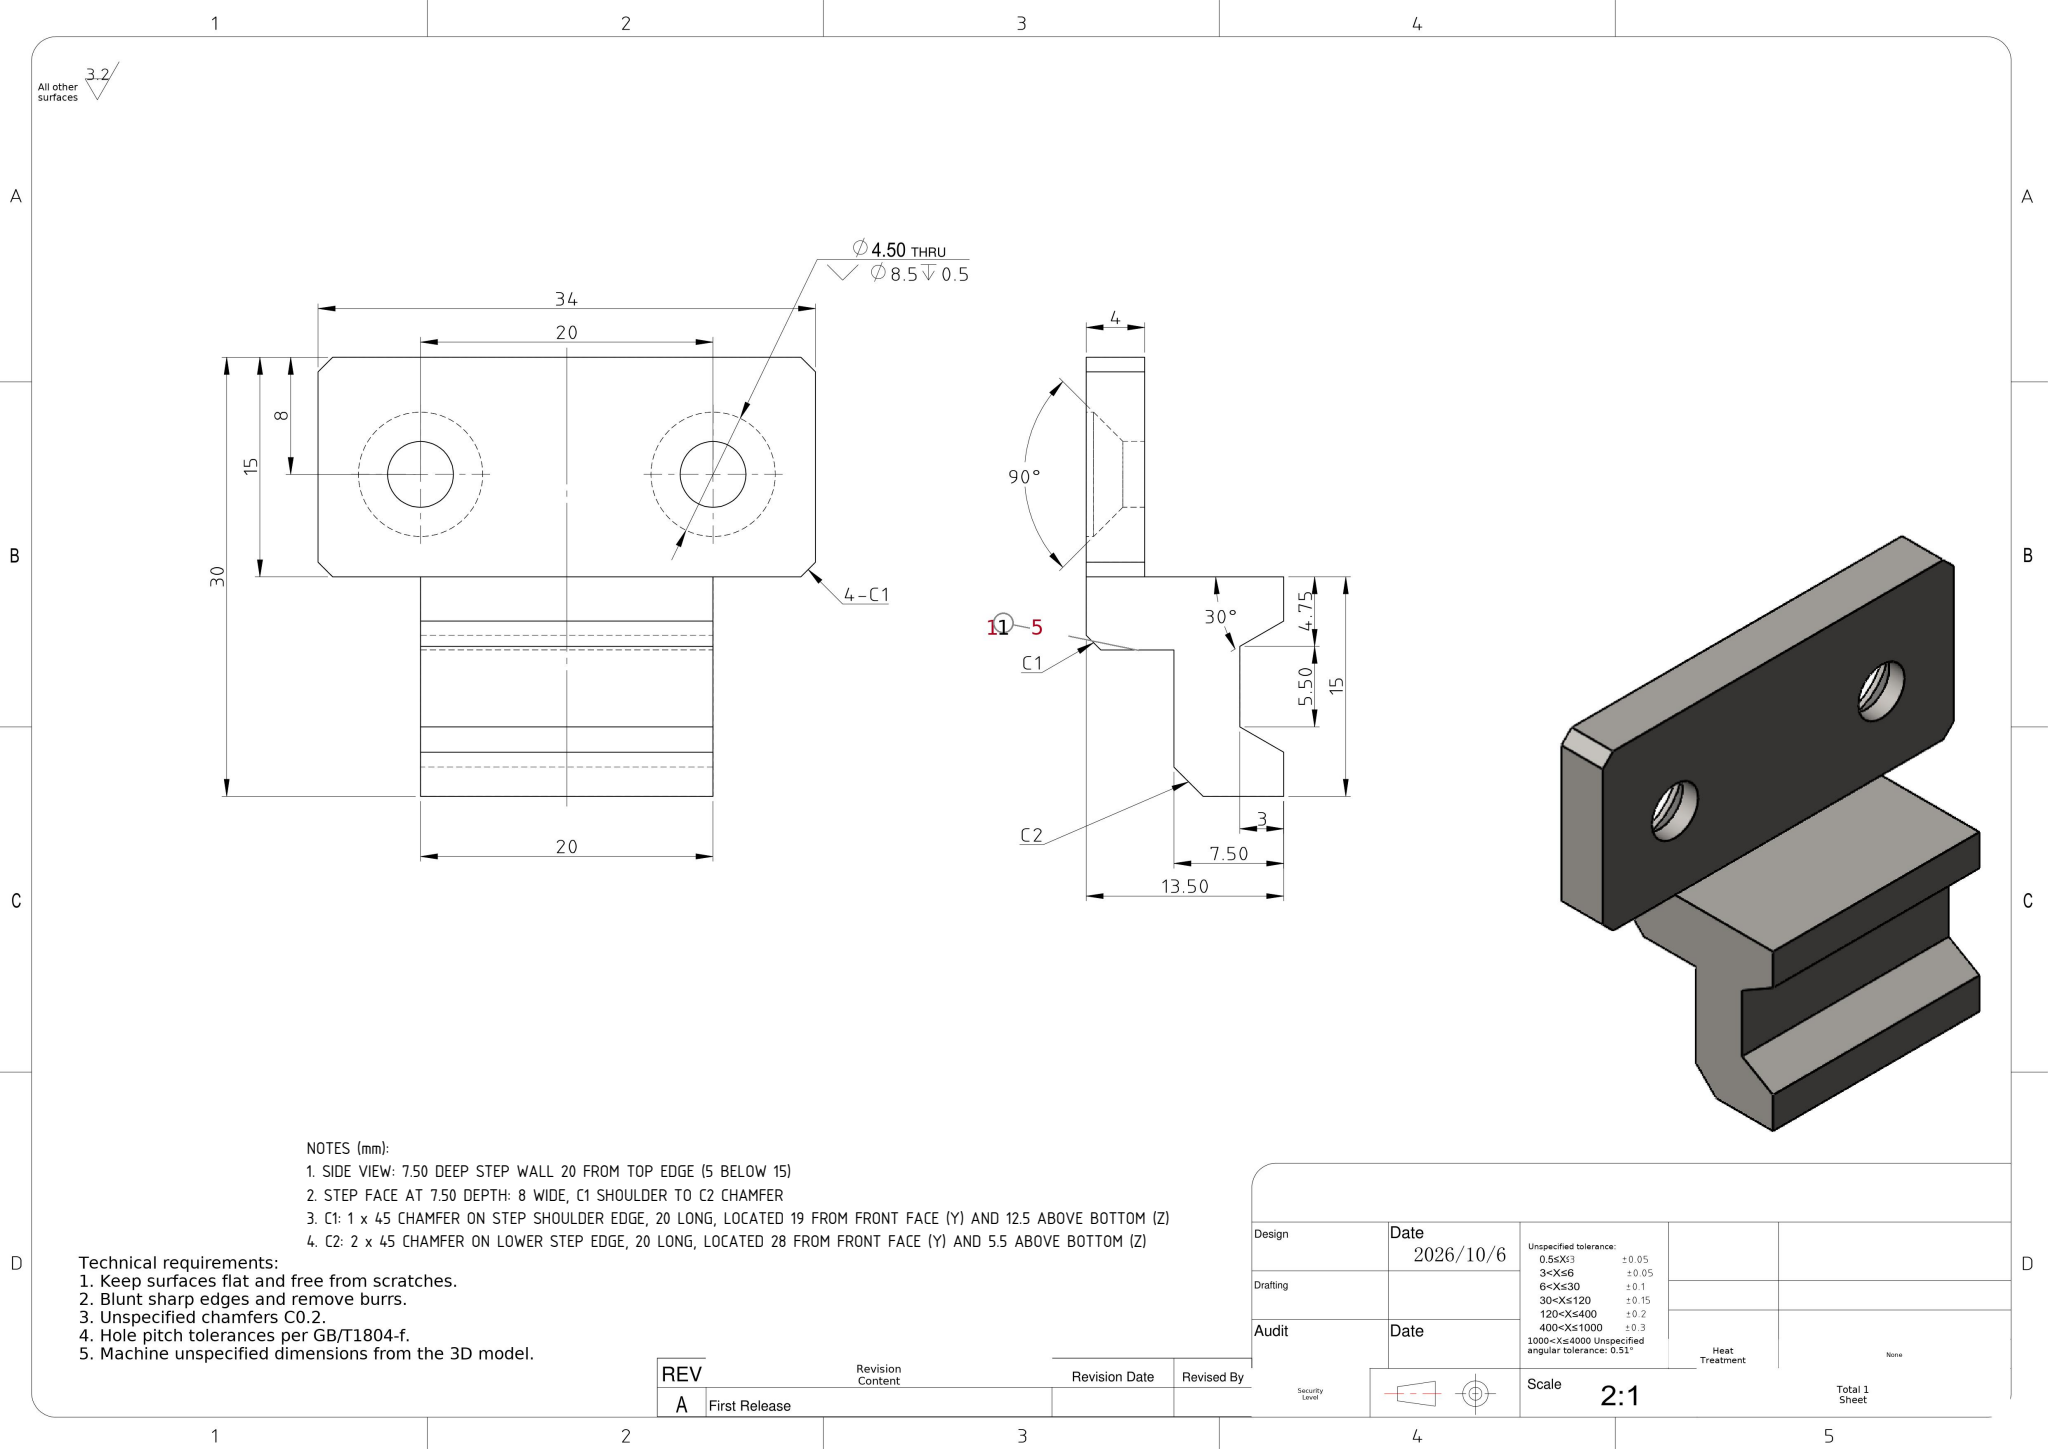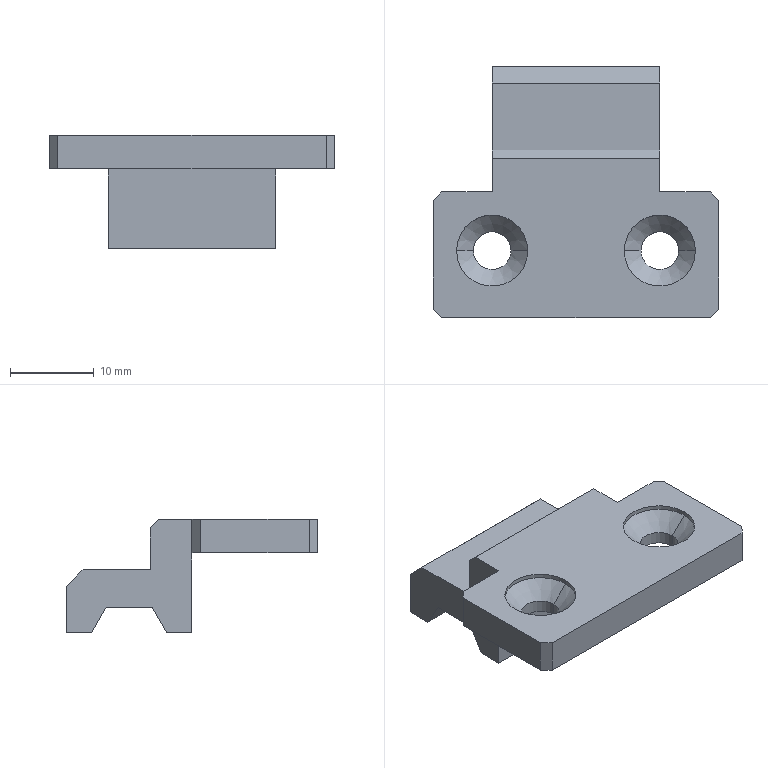Part | SolidWorks | mm | 1 solid | 36 faces | box 34 x 30 x 13.5 mm | volume 4157 mm3 | plane 24 | cylinder 8 | cone 4 | commonest cylinder face diameters 8.5 x4 4.5 x4
Drawing notes:
SIDE VIEW: 7.50 DEEP STEP WALL 20 FROM TOP EDGE (5 BELOW 15) | from the solid: Plane y=20, x[7,27], z[7.5,12.5]; plate top edge y=0, step datum line y=15
STEP FACE AT 7.50 DEPTH: 8 WIDE, C1 SHOULDER TO C2 CHAMFER | from the solid: Plane z=7.5 extent y[20,28] = 8 wide; C2 chamfer 2x2 at y[28,30], z[5.5,7.5]
C1: 1 x 45 CHAMFER ON STEP SHOULDER EDGE, 20 LONG, LOCATED 19 FROM FRONT FACE (Y) AND 12.5 ABOVE BOTTOM (Z) | from the solid: inclined_planes angle_to_xyz_axes [90,45,45], bbox_from [7.0,19.0,12.5], size [20.0,1.0,1.0]
C2: 2 x 45 CHAMFER ON LOWER STEP EDGE, 20 LONG, LOCATED 28 FROM FRONT FACE (Y) AND 5.5 ABOVE BOTTOM (Z) | from the solid: inclined_planes angle_to_xyz_axes [90,45,45], bbox_from [7.0,28.0,5.5], size [20.0,2.0,2.0]